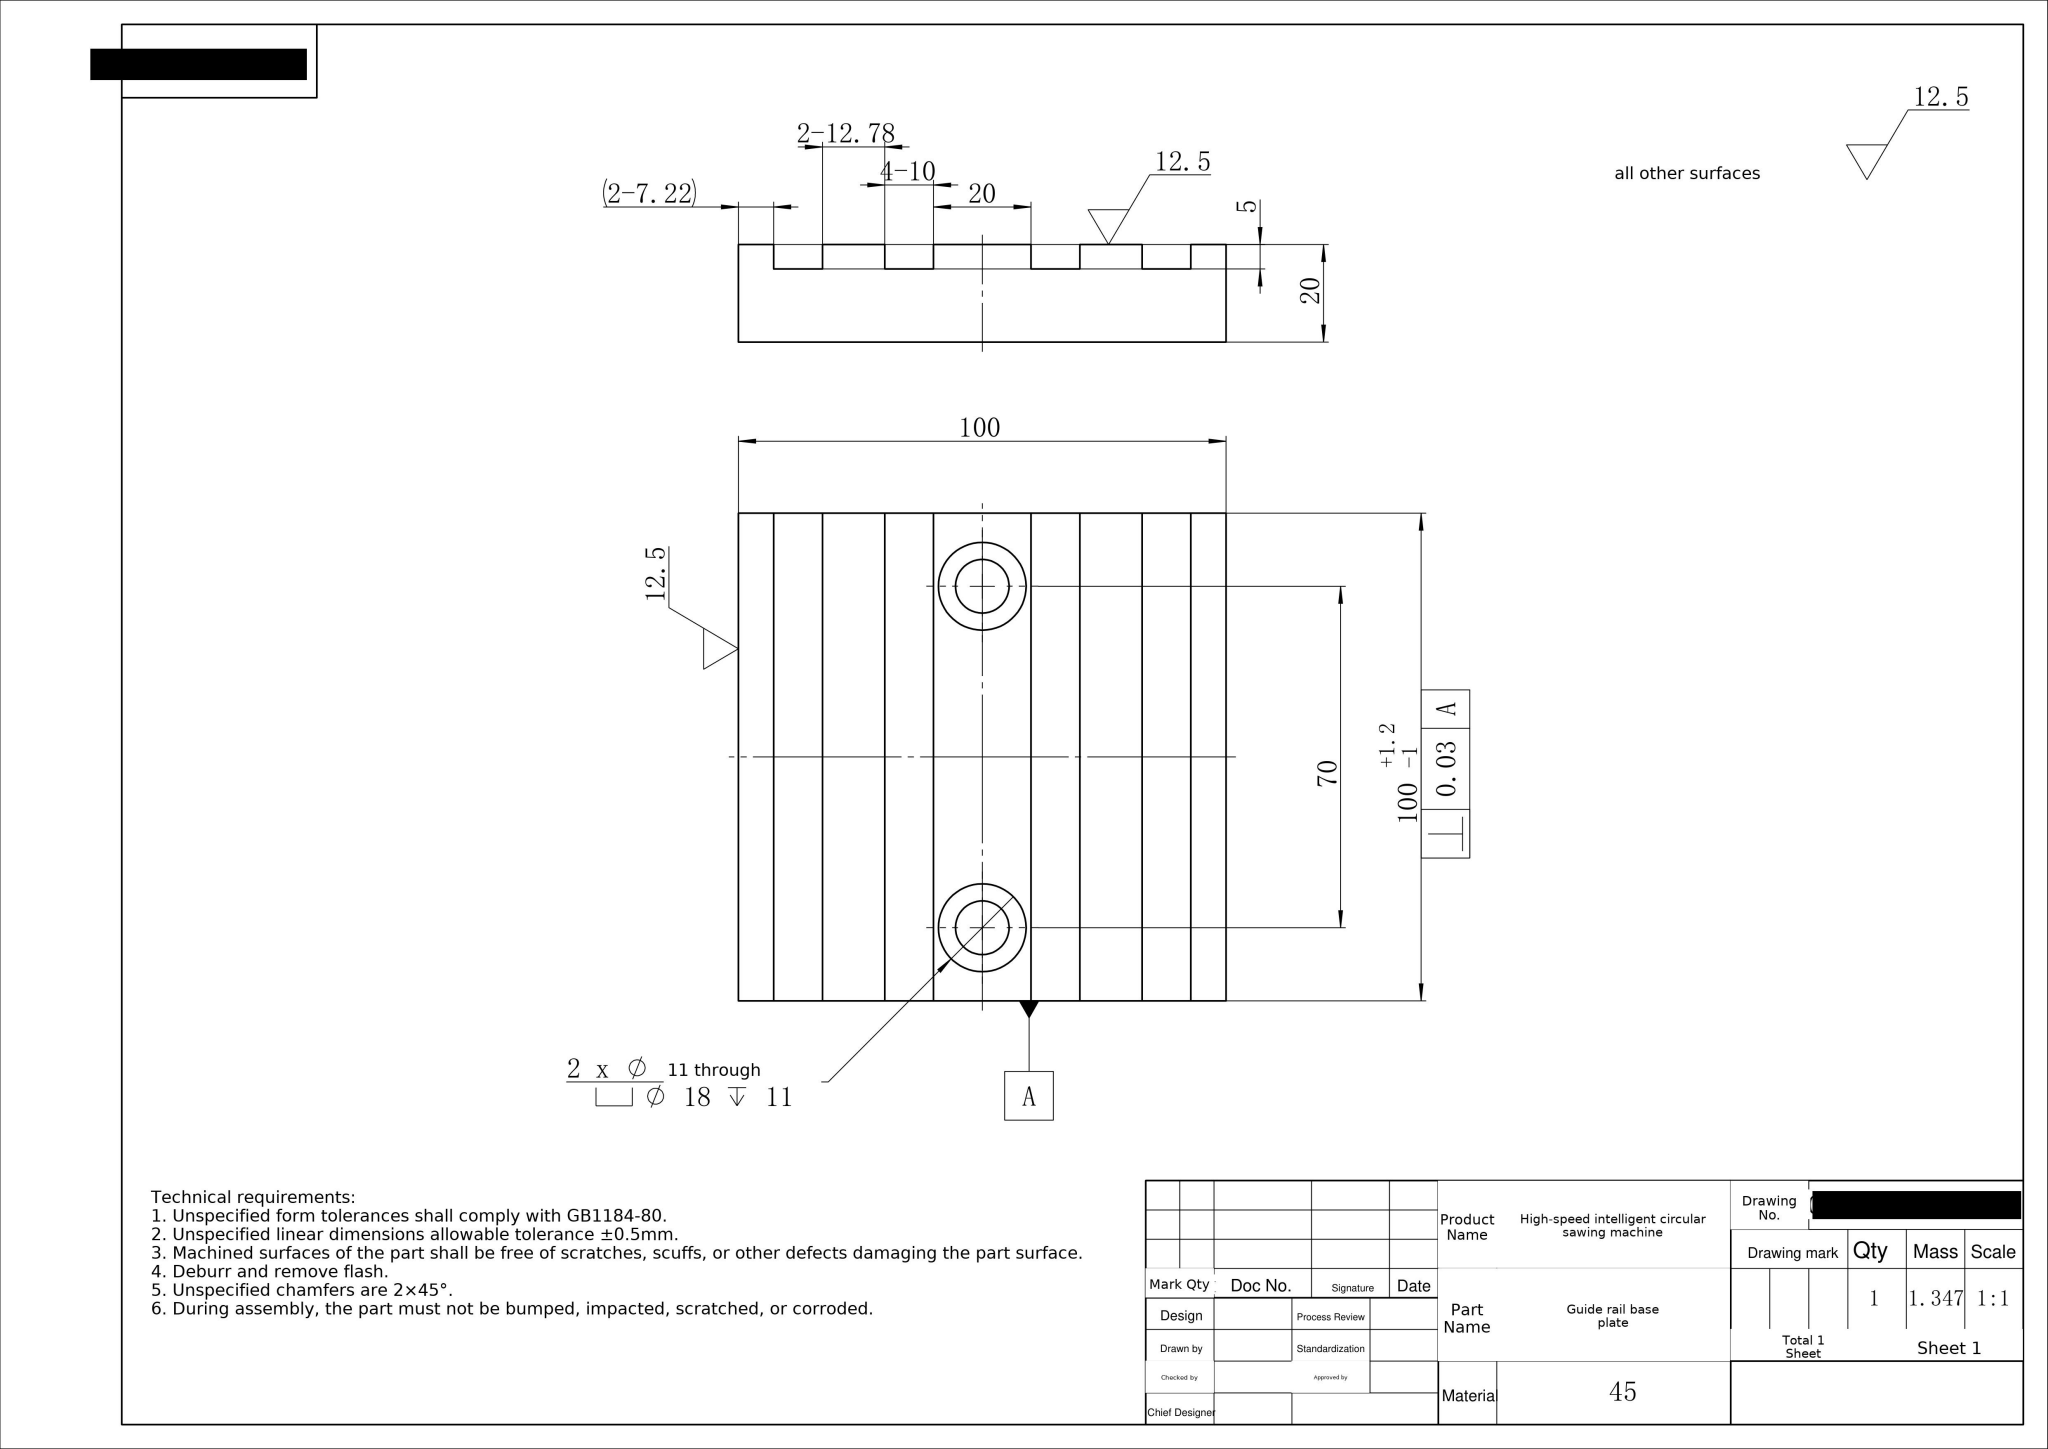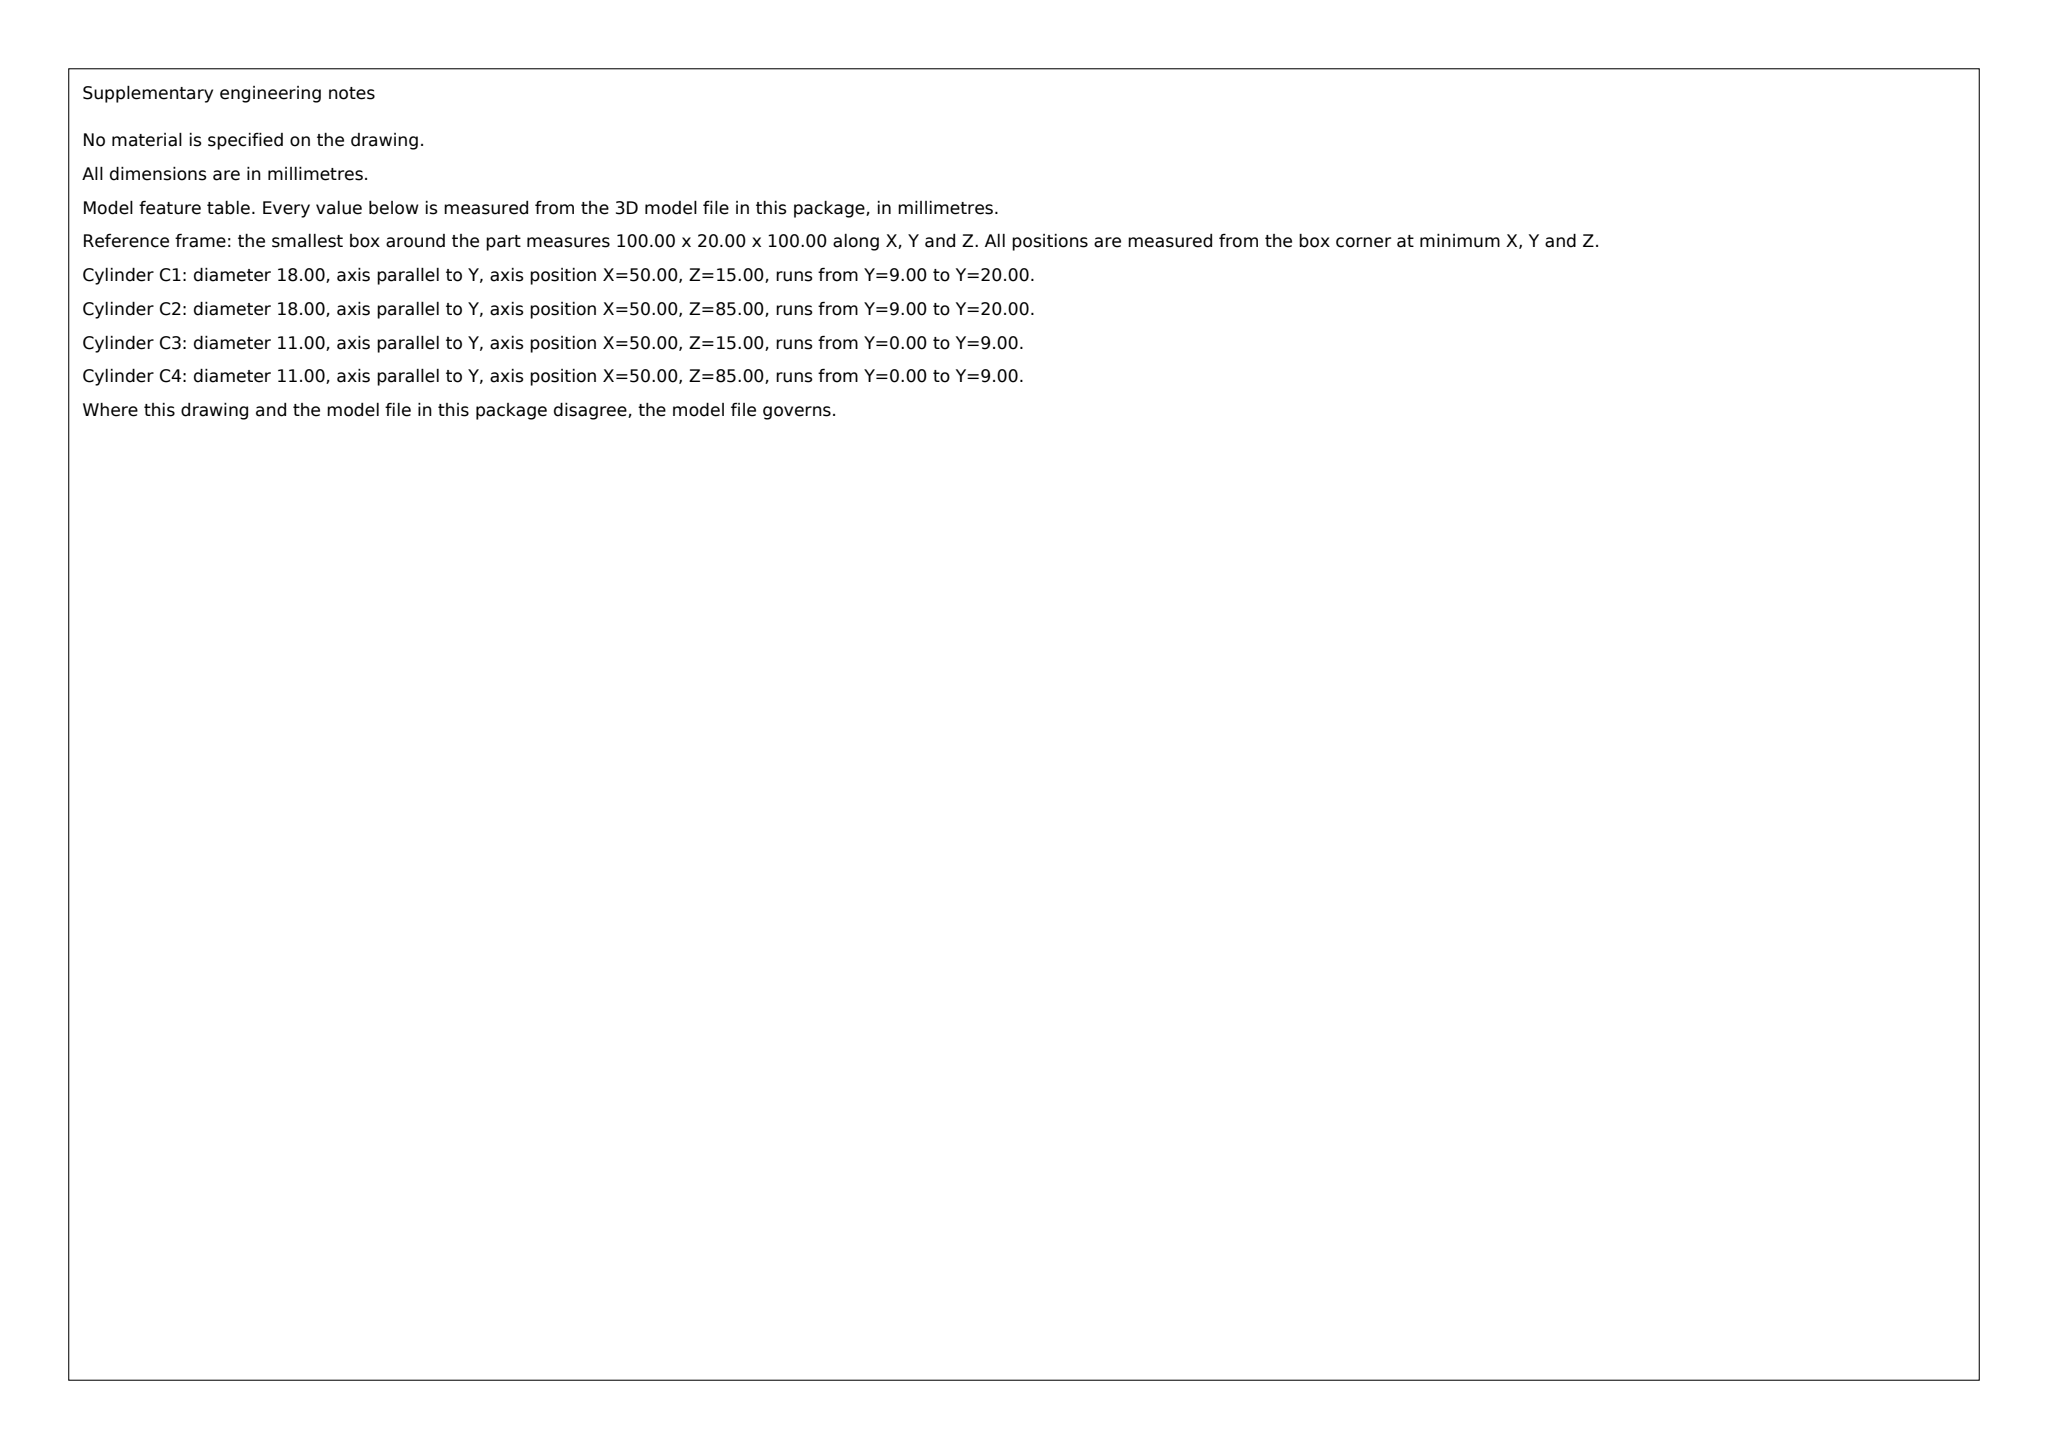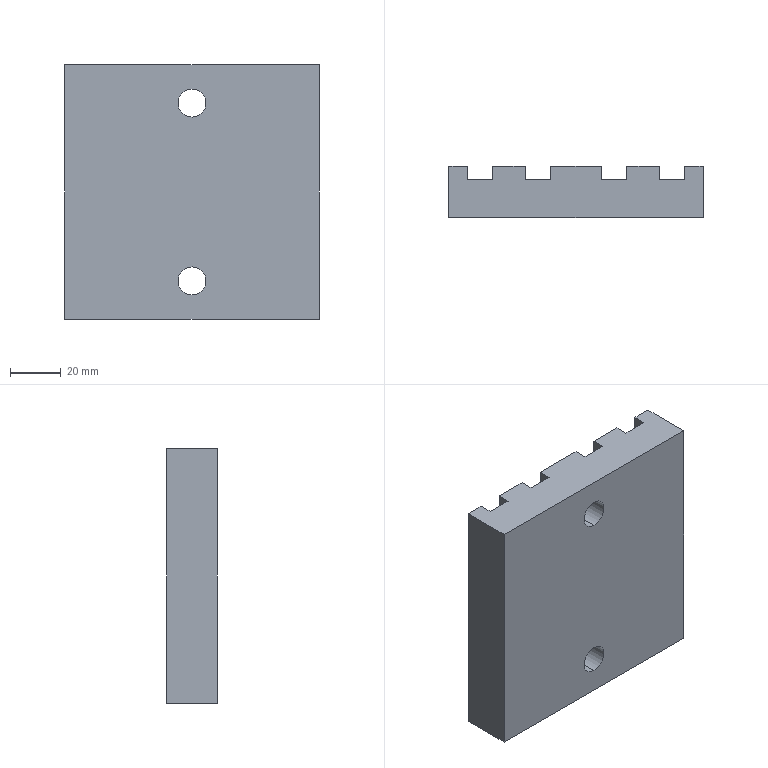Part | SolidWorks | mm | material 45 | 1 solid | 32 faces | box 100 x 20 x 100 mm | volume 172691 mm3 | plane 24 | cylinder 8 | commonest cylinder face diameters 18 x4 11 x4
build123d program:
from build123d import *

# Parameters (mm, degrees)
BOSS_EXTRUDE1_DEPTH                               = 100
CUT_EXTRUDE1_REACH                                = 115.578
SKETCH2_R                                         = 3.5
HOLE_SIZE_ACCORDING_TO_HEXAGON_SOCKET_D           = 11
HOLE_SIZE_ACCORDING_TO_HEXAGON_SOCKET_CBORE_D     = 18
HOLE_SIZE_ACCORDING_TO_HEXAGON_SOCKET_CBORE_DEPTH = 11


with BuildPart() as part:
    # Sketch1 → Boss-Extrude1 (new body)
    with BuildSketch(Plane.XY):
        Polygon((-50, 0), (50, 0), (50, 20), (42.78, 20), (42.78, 15), (32.78, 15), (32.78, 20), (20, 20), (20, 15), (10, 15), (10, 20), (-10, 20), (-10, 15), (-20, 15), (-20, 20), (-32.78, 20), (-32.78, 15), (-42.78, 15), (-42.78, 20), (-50, 20), align=None)
    extrude(amount=BOSS_EXTRUDE1_DEPTH)

    # Sketch2 → Cut-Extrude1 (cut, up to next)
    with BuildSketch(Plane.XZ, mode=Mode.PRIVATE) as cut_extrude1_sk1:
        with Locations(Location((0, 15, 0), (0, 0, 270))):
            Circle(SKETCH2_R)
    cut_extrude1_tool1 = extrude(cut_extrude1_sk1.sketch, amount=-CUT_EXTRUDE1_REACH, mode=Mode.PRIVATE) & part.part
    # Sketch2 → Cut-Extrude1 (cut, up to next)
    with BuildSketch(Plane.XZ, mode=Mode.PRIVATE) as cut_extrude1_sk2:
        with Locations(Location((0, 85, 0), (0, 0, 270))):
            Circle(SKETCH2_R)
    cut_extrude1_tool2 = extrude(cut_extrude1_sk2.sketch, amount=-CUT_EXTRUDE1_REACH, mode=Mode.PRIVATE) & part.part
    add(cut_extrude1_tool1.solids().sort_by_distance((0, 0, 15))[0], mode=Mode.SUBTRACT)
    add(cut_extrude1_tool2.solids().sort_by_distance((0, 0, 85))[0], mode=Mode.SUBTRACT)

    # Hole Size _according to_ Hexagon Socket (through all)
    with Locations(Plane(origin=(0, 20, 0), x_dir=(1, 0, 0), z_dir=(0, 1, 0))):
        with Locations((0, -15), (0, -85)):
            CounterBoreHole(HOLE_SIZE_ACCORDING_TO_HEXAGON_SOCKET_D / 2, HOLE_SIZE_ACCORDING_TO_HEXAGON_SOCKET_CBORE_D / 2, HOLE_SIZE_ACCORDING_TO_HEXAGON_SOCKET_CBORE_DEPTH)


solid = part.part